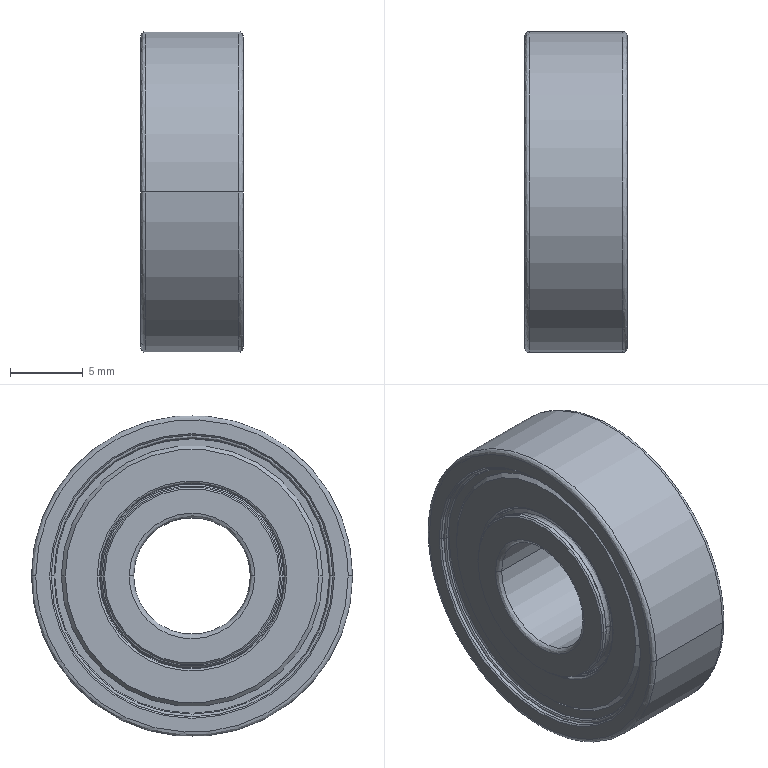Component | SolidWorks | BAF608ZZ-1 | 1 solid | 116 faces | volume 1819 mm3 | cone 44 | spline 32 | cylinder 28 | plane 12 | commonest cylinder face diameters 19.3 x4 12.73 x4 12.996 x4 17.9 x4 12.6 x4 12.2 x4 22 x2 8 x2